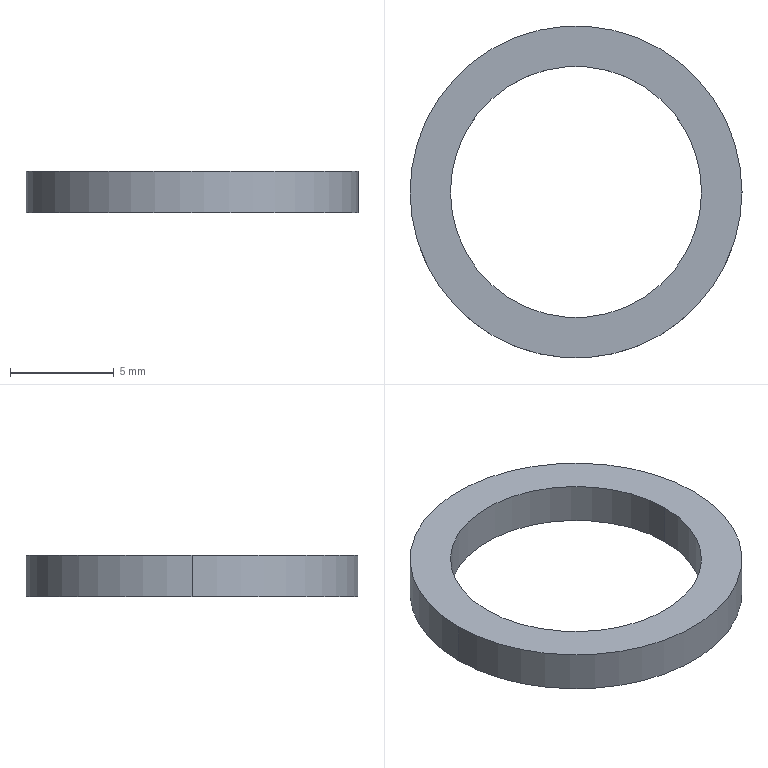Component | SolidWorks | TensioningWheel-2-1_XT-1-22-2-1 | 1 solid | 6 faces | box 16 x 16 x 2 mm | volume 172 mm3 | cylinder 4 | plane 2 | commonest cylinder face diameters 12.1 x2 16 x2
build123d program:
from build123d import *

# Parameters (mm, degrees)
SKETCH1_R           = 8
SKETCH1_R_2         = 6.05
BOSS_EXTRUDE1_DEPTH = 2


with BuildPart() as part:
    # Sketch1 → Boss-Extrude1 (new body)
    with BuildSketch(Plane.XY):
        Circle(SKETCH1_R)
        Circle(SKETCH1_R_2, mode=Mode.SUBTRACT)
    extrude(amount=BOSS_EXTRUDE1_DEPTH)


solid = part.part

# Placed as in the assembly
solid = solid.moved(Location((538.036, -118.615, -116), (0, 0, 0)))
STEP:
#1=COLOUR_RGB('',0.7922,0.8196,0.9333);
#2=FILL_AREA_STYLE_COLOUR('',#1);
#3=FILL_AREA_STYLE('',(#2));
#4=SURFACE_STYLE_FILL_AREA(#3);
#5=SURFACE_SIDE_STYLE('',(#4));
#6=SURFACE_STYLE_USAGE(.BOTH.,#5);
#7=PRESENTATION_STYLE_ASSIGNMENT((#6));
#8=CARTESIAN_POINT('',(20.944,-4.67,-4.488));
#9=VERTEX_POINT('',#8);
#10=CARTESIAN_POINT('',(21.421,-4.67,-4.488));
#11=VERTEX_POINT('',#10);
#12=CARTESIAN_POINT('',(21.183,-4.67,-4.488));
#13=DIRECTION('',(0.,0.,1.));
#14=DIRECTION('',(1.,0.,0.));
#15=AXIS2_PLACEMENT_3D('',#12,#13,#14);
#16=CIRCLE('',#15,0.2382);
#17=EDGE_CURVE('',#9,#11,#16,.T.);
#18=ORIENTED_EDGE('',*,*,#17,.T.);
#19=CARTESIAN_POINT('',(21.421,-4.67,-4.567));
#20=VERTEX_POINT('',#19);
#21=CARTESIAN_POINT('',(21.421,-4.67,-4.488));
#22=DIRECTION('',(0.,0.,-1.));
#23=VECTOR('',#22,39.37);
#24=LINE('',#21,#23);
#25=EDGE_CURVE('',#11,#20,#24,.T.);
#26=ORIENTED_EDGE('',*,*,#25,.T.);
#27=CARTESIAN_POINT('',(20.944,-4.67,-4.567));
#28=VERTEX_POINT('',#27);
#29=CARTESIAN_POINT('',(21.183,-4.67,-4.567));
#30=DIRECTION('',(0.,0.,1.));
#31=DIRECTION('',(1.,0.,0.));
#32=AXIS2_PLACEMENT_3D('',#29,#30,#31);
#33=CIRCLE('',#32,0.2382);
#34=EDGE_CURVE('',#28,#20,#33,.T.);
#35=ORIENTED_EDGE('',*,*,#34,.F.);
#36=CARTESIAN_POINT('',(20.944,-4.67,-4.488));
#37=DIRECTION('',(0.,0.,-1.));
#38=VECTOR('',#37,39.37);
#39=LINE('',#36,#38);
#40=EDGE_CURVE('',#9,#28,#39,.T.);
#41=ORIENTED_EDGE('',*,*,#40,.F.);
#42=EDGE_LOOP('',(#18,#26,#35,#41));
#43=FACE_OUTER_BOUND('',#42,.T.);
#44=CARTESIAN_POINT('',(21.183,-4.67,-4.488));
#45=DIRECTION('',(0.,0.,-1.));
#46=DIRECTION('',(-1.,0.,0.));
#47=AXIS2_PLACEMENT_3D('',#44,#45,#46);
#48=CYLINDRICAL_SURFACE('',#47,0.2382);
#49=ADVANCED_FACE('',(#43),#48,.F.);
#50=CARTESIAN_POINT('',(21.497,-4.67,-4.488));
#51=VERTEX_POINT('',#50);
#52=CARTESIAN_POINT('',(20.868,-4.67,-4.488));
#53=VERTEX_POINT('',#52);
#54=CARTESIAN_POINT('',(21.183,-4.67,-4.488));
#55=DIRECTION('',(0.,0.,1.));
#56=DIRECTION('',(1.,0.,0.));
#57=AXIS2_PLACEMENT_3D('',#54,#55,#56);
#58=CIRCLE('',#57,0.315);
#59=EDGE_CURVE('',#51,#53,#58,.T.);
#60=ORIENTED_EDGE('',*,*,#59,.F.);
#61=CARTESIAN_POINT('',(21.497,-4.67,-4.567));
#62=VERTEX_POINT('',#61);
#63=CARTESIAN_POINT('',(21.497,-4.67,-4.488));
#64=DIRECTION('',(0.,0.,-1.));
#65=VECTOR('',#64,39.37);
#66=LINE('',#63,#65);
#67=EDGE_CURVE('',#51,#62,#66,.T.);
#68=ORIENTED_EDGE('',*,*,#67,.T.);
#69=CARTESIAN_POINT('',(20.868,-4.67,-4.567));
#70=VERTEX_POINT('',#69);
#71=CARTESIAN_POINT('',(21.183,-4.67,-4.567));
#72=DIRECTION('',(0.,0.,1.));
#73=DIRECTION('',(1.,0.,0.));
#74=AXIS2_PLACEMENT_3D('',#71,#72,#73);
#75=CIRCLE('',#74,0.315);
#76=EDGE_CURVE('',#62,#70,#75,.T.);
#77=ORIENTED_EDGE('',*,*,#76,.T.);
#78=CARTESIAN_POINT('',(20.868,-4.67,-4.488));
#79=DIRECTION('',(0.,0.,-1.));
#80=VECTOR('',#79,39.37);
#81=LINE('',#78,#80);
#82=EDGE_CURVE('',#53,#70,#81,.T.);
#83=ORIENTED_EDGE('',*,*,#82,.F.);
#84=EDGE_LOOP('',(#60,#68,#77,#83));
#85=FACE_OUTER_BOUND('',#84,.T.);
#86=CARTESIAN_POINT('',(21.183,-4.67,-4.488));
#87=DIRECTION('',(0.,0.,-1.));
#88=DIRECTION('',(-1.,0.,0.));
#89=AXIS2_PLACEMENT_3D('',#86,#87,#88);
#90=CYLINDRICAL_SURFACE('',#89,0.315);
#91=ADVANCED_FACE('',(#85),#90,.T.);
#92=CARTESIAN_POINT('',(21.183,-4.67,-4.488));
#93=DIRECTION('',(0.,0.,1.));
#94=DIRECTION('',(1.,0.,0.));
#95=AXIS2_PLACEMENT_3D('',#92,#93,#94);
#96=CIRCLE('',#95,0.315);
#97=EDGE_CURVE('',#53,#51,#96,.T.);
#98=ORIENTED_EDGE('',*,*,#97,.T.);
#99=ORIENTED_EDGE('',*,*,#59,.T.);
#100=EDGE_LOOP('',(#98,#99));
#101=FACE_OUTER_BOUND('',#100,.T.);
#102=ORIENTED_EDGE('',*,*,#17,.F.);
#103=CARTESIAN_POINT('',(21.183,-4.67,-4.488));
#104=DIRECTION('',(0.,0.,1.));
#105=DIRECTION('',(1.,0.,0.));
#106=AXIS2_PLACEMENT_3D('',#103,#104,#105);
#107=CIRCLE('',#106,0.2382);
#108=EDGE_CURVE('',#11,#9,#107,.T.);
#109=ORIENTED_EDGE('',*,*,#108,.F.);
#110=EDGE_LOOP('',(#102,#109));
#111=FACE_BOUND('',#110,.T.);
#112=CARTESIAN_POINT('',(21.183,-4.67,-4.488));
#113=DIRECTION('',(0.,0.,1.));
#114=DIRECTION('',(1.,0.,0.));
#115=AXIS2_PLACEMENT_3D('',#112,#113,#114);
#116=PLANE('',#115);
#117=ADVANCED_FACE('',(#101,#111),#116,.T.);
#118=CARTESIAN_POINT('',(21.183,-4.67,-4.567));
#119=DIRECTION('',(0.,0.,1.));
#120=DIRECTION('',(1.,0.,0.));
#121=AXIS2_PLACEMENT_3D('',#118,#119,#120);
#122=CIRCLE('',#121,0.315);
#123=EDGE_CURVE('',#70,#62,#122,.T.);
#124=ORIENTED_EDGE('',*,*,#123,.F.);
#125=ORIENTED_EDGE('',*,*,#76,.F.);
#126=EDGE_LOOP('',(#124,#125));
#127=FACE_OUTER_BOUND('',#126,.T.);
#128=ORIENTED_EDGE('',*,*,#34,.T.);
#129=CARTESIAN_POINT('',(21.183,-4.67,-4.567));
#130=DIRECTION('',(0.,0.,1.));
#131=DIRECTION('',(1.,0.,0.));
#132=AXIS2_PLACEMENT_3D('',#129,#130,#131);
#133=CIRCLE('',#132,0.2382);
#134=EDGE_CURVE('',#20,#28,#133,.T.);
#135=ORIENTED_EDGE('',*,*,#134,.T.);
#136=EDGE_LOOP('',(#128,#135));
#137=FACE_BOUND('',#136,.T.);
#138=CARTESIAN_POINT('',(21.183,-4.67,-4.567));
#139=DIRECTION('',(0.,0.,1.));
#140=DIRECTION('',(1.,0.,0.));
#141=AXIS2_PLACEMENT_3D('',#138,#139,#140);
#142=PLANE('',#141);
#143=ADVANCED_FACE('',(#127,#137),#142,.F.);
#144=ORIENTED_EDGE('',*,*,#67,.F.);
#145=ORIENTED_EDGE('',*,*,#97,.F.);
#146=ORIENTED_EDGE('',*,*,#82,.T.);
#147=ORIENTED_EDGE('',*,*,#123,.T.);
#148=EDGE_LOOP('',(#144,#145,#146,#147));
#149=FACE_OUTER_BOUND('',#148,.T.);
#150=CARTESIAN_POINT('',(21.183,-4.67,-4.488));
#151=DIRECTION('',(0.,0.,-1.));
#152=DIRECTION('',(-1.,0.,0.));
#153=AXIS2_PLACEMENT_3D('',#150,#151,#152);
#154=CYLINDRICAL_SURFACE('',#153,0.315);
#155=ADVANCED_FACE('',(#149),#154,.T.);
#156=ORIENTED_EDGE('',*,*,#25,.F.);
#157=ORIENTED_EDGE('',*,*,#108,.T.);
#158=ORIENTED_EDGE('',*,*,#40,.T.);
#159=ORIENTED_EDGE('',*,*,#134,.F.);
#160=EDGE_LOOP('',(#156,#157,#158,#159));
#161=FACE_OUTER_BOUND('',#160,.T.);
#162=CARTESIAN_POINT('',(21.183,-4.67,-4.488));
#163=DIRECTION('',(0.,0.,-1.));
#164=DIRECTION('',(-1.,0.,0.));
#165=AXIS2_PLACEMENT_3D('',#162,#163,#164);
#166=CYLINDRICAL_SURFACE('',#165,0.2382);
#167=ADVANCED_FACE('',(#161),#166,.F.);
#168=CLOSED_SHELL('',(#49,#91,#117,#143,#155,#167));
#169=MANIFOLD_SOLID_BREP('',#168);
#170=STYLED_ITEM('',(#7),#169);
#171=(LENGTH_UNIT()NAMED_UNIT(*)SI_UNIT($,.METRE.));
#172=LENGTH_MEASURE_WITH_UNIT(LENGTH_MEASURE(0.0254),#171);
#173=DIMENSIONAL_EXPONENTS(1.,0.,0.,0.,0.,0.,0.);
#174=(CONVERSION_BASED_UNIT('',#172)LENGTH_UNIT()NAMED_UNIT(#173));
#175=UNCERTAINTY_MEASURE_WITH_UNIT(LENGTH_MEASURE(0.00001),#174,'','');
#176=(NAMED_UNIT(*)PLANE_ANGLE_UNIT()SI_UNIT($,.RADIAN.));
#177=(NAMED_UNIT(*)SI_UNIT($,.STERADIAN.)SOLID_ANGLE_UNIT());
#178=(GEOMETRIC_REPRESENTATION_CONTEXT(3)GLOBAL_UNCERTAINTY_ASSIGNED_CONTEXT((#175))GLOBAL_UNIT_ASSIGNED_CONTEXT((#174,#176,#177))REPRESENTATION_CONTEXT('',''));
#179=MECHANICAL_DESIGN_GEOMETRIC_PRESENTATION_REPRESENTATION('',(#170),#178);
#180=CARTESIAN_POINT('',(0.,0.,0.));
#181=DIRECTION('',(0.,0.,1.));
#182=DIRECTION('',(1.,0.,0.));
#183=AXIS2_PLACEMENT_3D('',#180,#181,#182);
#184=(LENGTH_UNIT()NAMED_UNIT(*)SI_UNIT($,.METRE.));
#185=LENGTH_MEASURE_WITH_UNIT(LENGTH_MEASURE(0.0254),#184);
#186=DIMENSIONAL_EXPONENTS(1.,0.,0.,0.,0.,0.,0.);
#187=(CONVERSION_BASED_UNIT('',#185)LENGTH_UNIT()NAMED_UNIT(#186));
#188=UNCERTAINTY_MEASURE_WITH_UNIT(LENGTH_MEASURE(0.00001),#187,'','');
#189=(NAMED_UNIT(*)PLANE_ANGLE_UNIT()SI_UNIT($,.RADIAN.));
#190=(NAMED_UNIT(*)SI_UNIT($,.STERADIAN.)SOLID_ANGLE_UNIT());
#191=(GEOMETRIC_REPRESENTATION_CONTEXT(3)GLOBAL_UNCERTAINTY_ASSIGNED_CONTEXT((#188))GLOBAL_UNIT_ASSIGNED_CONTEXT((#187,#189,#190))REPRESENTATION_CONTEXT('',''));
#192=ADVANCED_BREP_SHAPE_REPRESENTATION('',(#169,#183),#191);
#193=PRESENTATION_LAYER_ASSIGNMENT('','',(#170));